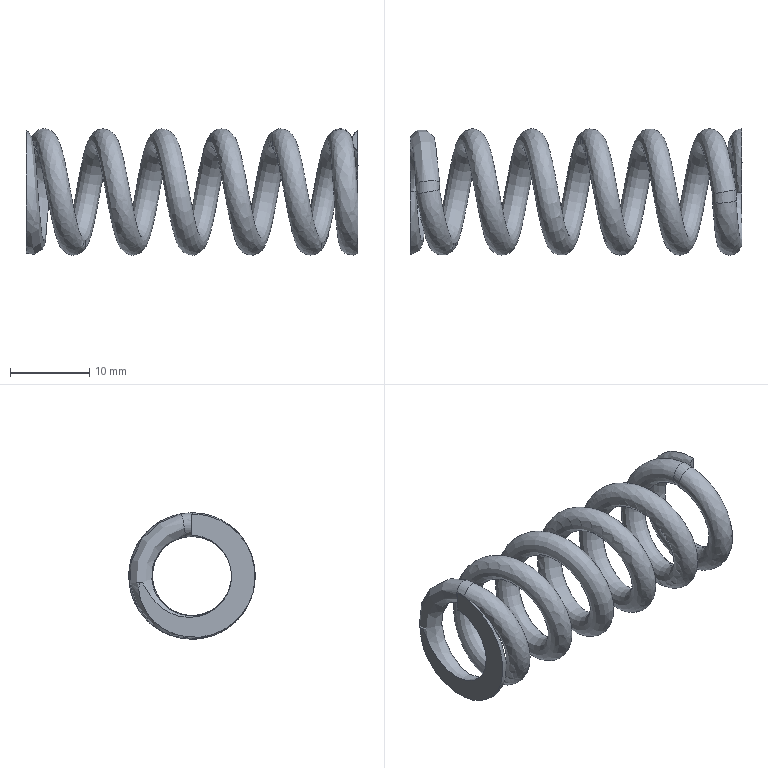Component | NX | SPRING | 1 solid | 9 faces | volume 1880 mm3 | spline 5 | plane 4